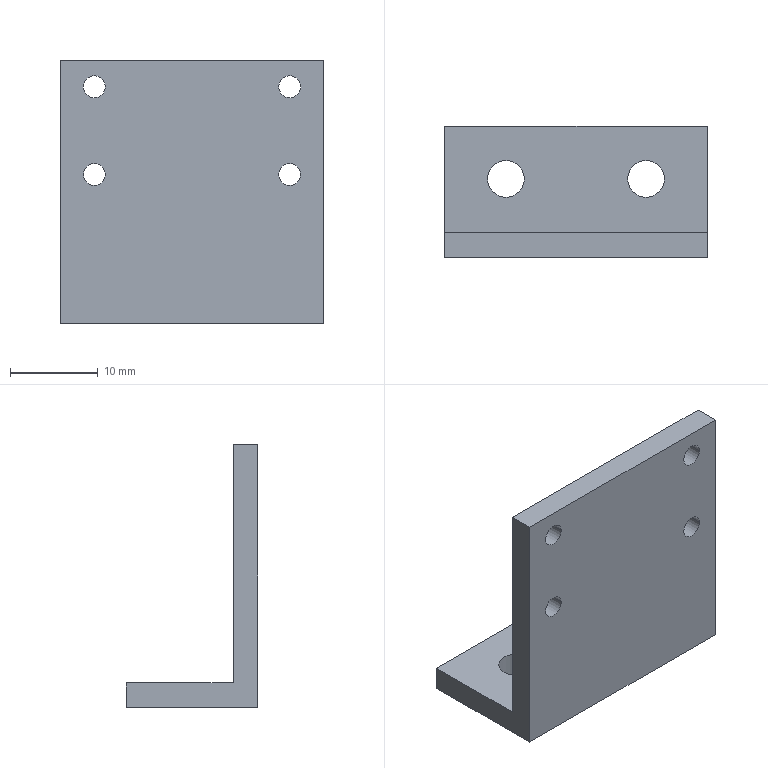Component | SolidWorks | 6G-DCSG-StopSwitchSeat-1 | 1 solid | 20 faces | box 30 x 15 x 30 mm | volume 3412 mm3 | cylinder 12 | plane 8 | commonest cylinder face diameters 2.5 x8 4.2 x4
build123d program:
from build123d import *

# Parameters (mm, degrees)
BOSS_EXTRUDE1_DEPTH = 15
SKETCH2_R           = 2.1
CUT_EXTRUDE1_DEPTH  = 10
M3_TAPPED_HOLE1_D   = 2.5


with BuildPart() as part:
    # Sketch1 → Boss-Extrude1 (new, symmetric)
    with BuildSketch(Plane.XY):
        Polygon((-15, 4.7), (12.2, 4.7), (12.2, -7.5), (15, -7.5), (15, 7.5), (-15, 7.5), align=None)
    extrude(amount=BOSS_EXTRUDE1_DEPTH, both=True)

    # Sketch2 → Cut-Extrude1 (cut)
    with BuildSketch(Plane.ZY.offset(-12.2)):
        with Locations((-8, -1.5)):
            Circle(SKETCH2_R)
        with Locations((8, -1.5)):
            Circle(SKETCH2_R)
    extrude(amount=-CUT_EXTRUDE1_DEPTH, mode=Mode.SUBTRACT)

    # M3 Tapped Hole1 (through all)
    with Locations(Plane(origin=(-12, 4.7, 11.15), x_dir=(0, 0, -1), z_dir=(0, -1, 0))):
        with Locations((0, 0), (0, 10), (22.3, 0), (22.3, 10)):
            Hole(M3_TAPPED_HOLE1_D / 2)


solid = part.part

# Placed as in the assembly
solid = solid.moved(Location((-162, 88.5, 15), (180, -90, 0)))
STEP:
#1=CARTESIAN_POINT('',(-6.866,3.189,1.063));
#2=VERTEX_POINT('',#1);
#3=CARTESIAN_POINT('',(-6.768,3.189,1.063));
#4=VERTEX_POINT('',#3);
#5=CARTESIAN_POINT('',(-6.817,3.189,1.063));
#6=DIRECTION('',(-0.,1.,0.));
#7=DIRECTION('',(1.,0.,0.));
#8=AXIS2_PLACEMENT_3D('',#5,#6,#7);
#9=CIRCLE('',#8,0.04921);
#10=EDGE_CURVE('',#2,#4,#9,.T.);
#11=ORIENTED_EDGE('',*,*,#10,.F.);
#12=CARTESIAN_POINT('',(-6.866,3.299,1.063));
#13=VERTEX_POINT('',#12);
#14=CARTESIAN_POINT('',(-6.866,3.299,1.063));
#15=DIRECTION('',(-0.,1.,0.));
#16=VECTOR('',#15,39.37);
#17=LINE('',#14,#16);
#18=EDGE_CURVE('',#2,#13,#17,.T.);
#19=ORIENTED_EDGE('',*,*,#18,.T.);
#20=CARTESIAN_POINT('',(-6.768,3.299,1.063));
#21=VERTEX_POINT('',#20);
#22=CARTESIAN_POINT('',(-6.817,3.299,1.063));
#23=DIRECTION('',(-0.,1.,0.));
#24=DIRECTION('',(1.,0.,0.));
#25=AXIS2_PLACEMENT_3D('',#22,#23,#24);
#26=CIRCLE('',#25,0.04921);
#27=EDGE_CURVE('',#13,#21,#26,.T.);
#28=ORIENTED_EDGE('',*,*,#27,.T.);
#29=CARTESIAN_POINT('',(-6.768,3.299,1.063));
#30=DIRECTION('',(-0.,1.,0.));
#31=VECTOR('',#30,39.37);
#32=LINE('',#29,#31);
#33=EDGE_CURVE('',#4,#21,#32,.T.);
#34=ORIENTED_EDGE('',*,*,#33,.F.);
#35=EDGE_LOOP('',(#11,#19,#28,#34));
#36=FACE_OUTER_BOUND('',#35,.T.);
#37=CARTESIAN_POINT('',(-6.817,3.299,1.063));
#38=DIRECTION('',(-0.,1.,0.));
#39=DIRECTION('',(1.,0.,0.));
#40=AXIS2_PLACEMENT_3D('',#37,#38,#39);
#41=CYLINDRICAL_SURFACE('',#40,0.04921);
#42=ADVANCED_FACE('',(#36),#41,.F.);
#43=CARTESIAN_POINT('',(-6.866,3.189,0.6693));
#44=VERTEX_POINT('',#43);
#45=CARTESIAN_POINT('',(-6.768,3.189,0.6693));
#46=VERTEX_POINT('',#45);
#47=CARTESIAN_POINT('',(-6.817,3.189,0.6693));
#48=DIRECTION('',(-0.,1.,0.));
#49=DIRECTION('',(1.,0.,0.));
#50=AXIS2_PLACEMENT_3D('',#47,#48,#49);
#51=CIRCLE('',#50,0.04921);
#52=EDGE_CURVE('',#44,#46,#51,.T.);
#53=ORIENTED_EDGE('',*,*,#52,.F.);
#54=CARTESIAN_POINT('',(-6.866,3.299,0.6693));
#55=VERTEX_POINT('',#54);
#56=CARTESIAN_POINT('',(-6.866,3.299,0.6693));
#57=DIRECTION('',(-0.,1.,0.));
#58=VECTOR('',#57,39.37);
#59=LINE('',#56,#58);
#60=EDGE_CURVE('',#44,#55,#59,.T.);
#61=ORIENTED_EDGE('',*,*,#60,.T.);
#62=CARTESIAN_POINT('',(-6.768,3.299,0.6693));
#63=VERTEX_POINT('',#62);
#64=CARTESIAN_POINT('',(-6.817,3.299,0.6693));
#65=DIRECTION('',(-0.,1.,0.));
#66=DIRECTION('',(1.,0.,0.));
#67=AXIS2_PLACEMENT_3D('',#64,#65,#66);
#68=CIRCLE('',#67,0.04921);
#69=EDGE_CURVE('',#55,#63,#68,.T.);
#70=ORIENTED_EDGE('',*,*,#69,.T.);
#71=CARTESIAN_POINT('',(-6.768,3.299,0.6693));
#72=DIRECTION('',(-0.,1.,0.));
#73=VECTOR('',#72,39.37);
#74=LINE('',#71,#73);
#75=EDGE_CURVE('',#46,#63,#74,.T.);
#76=ORIENTED_EDGE('',*,*,#75,.F.);
#77=EDGE_LOOP('',(#53,#61,#70,#76));
#78=FACE_OUTER_BOUND('',#77,.T.);
#79=CARTESIAN_POINT('',(-6.817,3.299,0.6693));
#80=DIRECTION('',(-0.,1.,0.));
#81=DIRECTION('',(1.,0.,0.));
#82=AXIS2_PLACEMENT_3D('',#79,#80,#81);
#83=CYLINDRICAL_SURFACE('',#82,0.04921);
#84=ADVANCED_FACE('',(#78),#83,.F.);
#85=CARTESIAN_POINT('',(-5.988,3.189,1.063));
#86=VERTEX_POINT('',#85);
#87=CARTESIAN_POINT('',(-5.89,3.189,1.063));
#88=VERTEX_POINT('',#87);
#89=CARTESIAN_POINT('',(-5.939,3.189,1.063));
#90=DIRECTION('',(-0.,1.,0.));
#91=DIRECTION('',(1.,0.,0.));
#92=AXIS2_PLACEMENT_3D('',#89,#90,#91);
#93=CIRCLE('',#92,0.04921);
#94=EDGE_CURVE('',#86,#88,#93,.T.);
#95=ORIENTED_EDGE('',*,*,#94,.F.);
#96=CARTESIAN_POINT('',(-5.988,3.299,1.063));
#97=VERTEX_POINT('',#96);
#98=CARTESIAN_POINT('',(-5.988,3.299,1.063));
#99=DIRECTION('',(-0.,1.,0.));
#100=VECTOR('',#99,39.37);
#101=LINE('',#98,#100);
#102=EDGE_CURVE('',#86,#97,#101,.T.);
#103=ORIENTED_EDGE('',*,*,#102,.T.);
#104=CARTESIAN_POINT('',(-5.89,3.299,1.063));
#105=VERTEX_POINT('',#104);
#106=CARTESIAN_POINT('',(-5.939,3.299,1.063));
#107=DIRECTION('',(-0.,1.,0.));
#108=DIRECTION('',(1.,0.,0.));
#109=AXIS2_PLACEMENT_3D('',#106,#107,#108);
#110=CIRCLE('',#109,0.04921);
#111=EDGE_CURVE('',#97,#105,#110,.T.);
#112=ORIENTED_EDGE('',*,*,#111,.T.);
#113=CARTESIAN_POINT('',(-5.89,3.299,1.063));
#114=DIRECTION('',(-0.,1.,0.));
#115=VECTOR('',#114,39.37);
#116=LINE('',#113,#115);
#117=EDGE_CURVE('',#88,#105,#116,.T.);
#118=ORIENTED_EDGE('',*,*,#117,.F.);
#119=EDGE_LOOP('',(#95,#103,#112,#118));
#120=FACE_OUTER_BOUND('',#119,.T.);
#121=CARTESIAN_POINT('',(-5.939,3.299,1.063));
#122=DIRECTION('',(-0.,1.,0.));
#123=DIRECTION('',(1.,0.,0.));
#124=AXIS2_PLACEMENT_3D('',#121,#122,#123);
#125=CYLINDRICAL_SURFACE('',#124,0.04921);
#126=ADVANCED_FACE('',(#120),#125,.F.);
#127=CARTESIAN_POINT('',(-5.988,3.189,0.6693));
#128=VERTEX_POINT('',#127);
#129=CARTESIAN_POINT('',(-5.89,3.189,0.6693));
#130=VERTEX_POINT('',#129);
#131=CARTESIAN_POINT('',(-5.939,3.189,0.6693));
#132=DIRECTION('',(-0.,1.,0.));
#133=DIRECTION('',(1.,0.,0.));
#134=AXIS2_PLACEMENT_3D('',#131,#132,#133);
#135=CIRCLE('',#134,0.04921);
#136=EDGE_CURVE('',#128,#130,#135,.T.);
#137=ORIENTED_EDGE('',*,*,#136,.F.);
#138=CARTESIAN_POINT('',(-5.988,3.299,0.6693));
#139=VERTEX_POINT('',#138);
#140=CARTESIAN_POINT('',(-5.988,3.299,0.6693));
#141=DIRECTION('',(-0.,1.,0.));
#142=VECTOR('',#141,39.37);
#143=LINE('',#140,#142);
#144=EDGE_CURVE('',#128,#139,#143,.T.);
#145=ORIENTED_EDGE('',*,*,#144,.T.);
#146=CARTESIAN_POINT('',(-5.89,3.299,0.6693));
#147=VERTEX_POINT('',#146);
#148=CARTESIAN_POINT('',(-5.939,3.299,0.6693));
#149=DIRECTION('',(-0.,1.,0.));
#150=DIRECTION('',(1.,0.,0.));
#151=AXIS2_PLACEMENT_3D('',#148,#149,#150);
#152=CIRCLE('',#151,0.04921);
#153=EDGE_CURVE('',#139,#147,#152,.T.);
#154=ORIENTED_EDGE('',*,*,#153,.T.);
#155=CARTESIAN_POINT('',(-5.89,3.299,0.6693));
#156=DIRECTION('',(-0.,1.,0.));
#157=VECTOR('',#156,39.37);
#158=LINE('',#155,#157);
#159=EDGE_CURVE('',#130,#147,#158,.T.);
#160=ORIENTED_EDGE('',*,*,#159,.F.);
#161=EDGE_LOOP('',(#137,#145,#154,#160));
#162=FACE_OUTER_BOUND('',#161,.T.);
#163=CARTESIAN_POINT('',(-5.939,3.299,0.6693));
#164=DIRECTION('',(-0.,1.,0.));
#165=DIRECTION('',(1.,0.,0.));
#166=AXIS2_PLACEMENT_3D('',#163,#164,#165);
#167=CYLINDRICAL_SURFACE('',#166,0.04921);
#168=ADVANCED_FACE('',(#162),#167,.F.);
#169=CARTESIAN_POINT('',(-6.61,3.543,0.));
#170=VERTEX_POINT('',#169);
#171=CARTESIAN_POINT('',(-6.776,3.543,0.));
#172=VERTEX_POINT('',#171);
#173=CARTESIAN_POINT('',(-6.693,3.543,0.));
#174=DIRECTION('',(-0.,-0.,1.));
#175=DIRECTION('',(-1.,0.,0.));
#176=AXIS2_PLACEMENT_3D('',#173,#174,#175);
#177=CIRCLE('',#176,0.08268);
#178=EDGE_CURVE('',#170,#172,#177,.T.);
#179=ORIENTED_EDGE('',*,*,#178,.F.);
#180=CARTESIAN_POINT('',(-6.61,3.543,0.1102));
#181=VERTEX_POINT('',#180);
#182=CARTESIAN_POINT('',(-6.61,3.543,-0.2835));
#183=DIRECTION('',(-0.,-0.,1.));
#184=VECTOR('',#183,39.37);
#185=LINE('',#182,#184);
#186=EDGE_CURVE('',#170,#181,#185,.T.);
#187=ORIENTED_EDGE('',*,*,#186,.T.);
#188=CARTESIAN_POINT('',(-6.776,3.543,0.1102));
#189=VERTEX_POINT('',#188);
#190=CARTESIAN_POINT('',(-6.693,3.543,0.1102));
#191=DIRECTION('',(-0.,-0.,1.));
#192=DIRECTION('',(-1.,0.,0.));
#193=AXIS2_PLACEMENT_3D('',#190,#191,#192);
#194=CIRCLE('',#193,0.08268);
#195=EDGE_CURVE('',#181,#189,#194,.T.);
#196=ORIENTED_EDGE('',*,*,#195,.T.);
#197=CARTESIAN_POINT('',(-6.776,3.543,-0.2835));
#198=DIRECTION('',(-0.,-0.,1.));
#199=VECTOR('',#198,39.37);
#200=LINE('',#197,#199);
#201=EDGE_CURVE('',#172,#189,#200,.T.);
#202=ORIENTED_EDGE('',*,*,#201,.F.);
#203=EDGE_LOOP('',(#179,#187,#196,#202));
#204=FACE_OUTER_BOUND('',#203,.T.);
#205=CARTESIAN_POINT('',(-6.693,3.543,-0.2835));
#206=DIRECTION('',(-0.,-0.,1.));
#207=DIRECTION('',(-1.,0.,0.));
#208=AXIS2_PLACEMENT_3D('',#205,#206,#207);
#209=CYLINDRICAL_SURFACE('',#208,0.08268);
#210=ADVANCED_FACE('',(#204),#209,.F.);
#211=CARTESIAN_POINT('',(-5.98,3.543,0.));
#212=VERTEX_POINT('',#211);
#213=CARTESIAN_POINT('',(-6.146,3.543,0.));
#214=VERTEX_POINT('',#213);
#215=CARTESIAN_POINT('',(-6.063,3.543,0.));
#216=DIRECTION('',(-0.,-0.,1.));
#217=DIRECTION('',(-1.,0.,0.));
#218=AXIS2_PLACEMENT_3D('',#215,#216,#217);
#219=CIRCLE('',#218,0.08268);
#220=EDGE_CURVE('',#212,#214,#219,.T.);
#221=ORIENTED_EDGE('',*,*,#220,.F.);
#222=CARTESIAN_POINT('',(-5.98,3.543,0.1102));
#223=VERTEX_POINT('',#222);
#224=CARTESIAN_POINT('',(-5.98,3.543,-0.2835));
#225=DIRECTION('',(-0.,-0.,1.));
#226=VECTOR('',#225,39.37);
#227=LINE('',#224,#226);
#228=EDGE_CURVE('',#212,#223,#227,.T.);
#229=ORIENTED_EDGE('',*,*,#228,.T.);
#230=CARTESIAN_POINT('',(-6.146,3.543,0.1102));
#231=VERTEX_POINT('',#230);
#232=CARTESIAN_POINT('',(-6.063,3.543,0.1102));
#233=DIRECTION('',(-0.,-0.,1.));
#234=DIRECTION('',(-1.,0.,0.));
#235=AXIS2_PLACEMENT_3D('',#232,#233,#234);
#236=CIRCLE('',#235,0.08268);
#237=EDGE_CURVE('',#223,#231,#236,.T.);
#238=ORIENTED_EDGE('',*,*,#237,.T.);
#239=CARTESIAN_POINT('',(-6.146,3.543,-0.2835));
#240=DIRECTION('',(-0.,-0.,1.));
#241=VECTOR('',#240,39.37);
#242=LINE('',#239,#241);
#243=EDGE_CURVE('',#214,#231,#242,.T.);
#244=ORIENTED_EDGE('',*,*,#243,.F.);
#245=EDGE_LOOP('',(#221,#229,#238,#244));
#246=FACE_OUTER_BOUND('',#245,.T.);
#247=CARTESIAN_POINT('',(-6.063,3.543,-0.2835));
#248=DIRECTION('',(-0.,-0.,1.));
#249=DIRECTION('',(-1.,0.,0.));
#250=AXIS2_PLACEMENT_3D('',#247,#248,#249);
#251=CYLINDRICAL_SURFACE('',#250,0.08268);
#252=ADVANCED_FACE('',(#246),#251,.F.);
#253=CARTESIAN_POINT('',(-6.693,3.543,0.));
#254=DIRECTION('',(-0.,-0.,1.));
#255=DIRECTION('',(-1.,0.,0.));
#256=AXIS2_PLACEMENT_3D('',#253,#254,#255);
#257=CIRCLE('',#256,0.08268);
#258=EDGE_CURVE('',#172,#170,#257,.T.);
#259=ORIENTED_EDGE('',*,*,#258,.T.);
#260=ORIENTED_EDGE('',*,*,#178,.T.);
#261=EDGE_LOOP('',(#259,#260));
#262=FACE_BOUND('',#261,.T.);
#263=CARTESIAN_POINT('',(-6.063,3.543,0.));
#264=DIRECTION('',(-0.,-0.,1.));
#265=DIRECTION('',(-1.,0.,0.));
#266=AXIS2_PLACEMENT_3D('',#263,#264,#265);
#267=CIRCLE('',#266,0.08268);
#268=EDGE_CURVE('',#214,#212,#267,.T.);
#269=ORIENTED_EDGE('',*,*,#268,.T.);
#270=ORIENTED_EDGE('',*,*,#220,.T.);
#271=EDGE_LOOP('',(#269,#270));
#272=FACE_BOUND('',#271,.T.);
#273=CARTESIAN_POINT('',(-5.787,3.78,0.));
#274=VERTEX_POINT('',#273);
#275=CARTESIAN_POINT('',(-5.787,3.189,0.));
#276=VERTEX_POINT('',#275);
#277=CARTESIAN_POINT('',(-5.787,3.78,0.));
#278=DIRECTION('',(0.,-1.,-0.));
#279=VECTOR('',#278,39.37);
#280=LINE('',#277,#279);
#281=EDGE_CURVE('',#274,#276,#280,.T.);
#282=ORIENTED_EDGE('',*,*,#281,.T.);
#283=CARTESIAN_POINT('',(-6.969,3.189,0.));
#284=VERTEX_POINT('',#283);
#285=CARTESIAN_POINT('',(-6.969,3.189,0.));
#286=DIRECTION('',(1.,0.,0.));
#287=VECTOR('',#286,39.37);
#288=LINE('',#285,#287);
#289=EDGE_CURVE('',#284,#276,#288,.T.);
#290=ORIENTED_EDGE('',*,*,#289,.F.);
#291=CARTESIAN_POINT('',(-6.969,3.78,0.));
#292=VERTEX_POINT('',#291);
#293=CARTESIAN_POINT('',(-6.969,3.78,0.));
#294=DIRECTION('',(0.,-1.,-0.));
#295=VECTOR('',#294,39.37);
#296=LINE('',#293,#295);
#297=EDGE_CURVE('',#292,#284,#296,.T.);
#298=ORIENTED_EDGE('',*,*,#297,.F.);
#299=CARTESIAN_POINT('',(-6.969,3.78,0.));
#300=DIRECTION('',(1.,0.,0.));
#301=VECTOR('',#300,39.37);
#302=LINE('',#299,#301);
#303=EDGE_CURVE('',#292,#274,#302,.T.);
#304=ORIENTED_EDGE('',*,*,#303,.T.);
#305=EDGE_LOOP('',(#282,#290,#298,#304));
#306=FACE_OUTER_BOUND('',#305,.T.);
#307=CARTESIAN_POINT('',(-6.969,3.78,0.));
#308=DIRECTION('',(0.,-0.,1.));
#309=DIRECTION('',(-1.,-0.,0.));
#310=AXIS2_PLACEMENT_3D('',#307,#308,#309);
#311=PLANE('',#310);
#312=ADVANCED_FACE('',(#262,#272,#306),#311,.F.);
#313=CARTESIAN_POINT('',(-6.817,3.189,1.063));
#314=DIRECTION('',(-0.,1.,0.));
#315=DIRECTION('',(1.,0.,0.));
#316=AXIS2_PLACEMENT_3D('',#313,#314,#315);
#317=CIRCLE('',#316,0.04921);
#318=EDGE_CURVE('',#4,#2,#317,.T.);
#319=ORIENTED_EDGE('',*,*,#318,.T.);
#320=ORIENTED_EDGE('',*,*,#10,.T.);
#321=EDGE_LOOP('',(#319,#320));
#322=FACE_BOUND('',#321,.T.);
#323=CARTESIAN_POINT('',(-6.817,3.189,0.6693));
#324=DIRECTION('',(-0.,1.,0.));
#325=DIRECTION('',(1.,0.,0.));
#326=AXIS2_PLACEMENT_3D('',#323,#324,#325);
#327=CIRCLE('',#326,0.04921);
#328=EDGE_CURVE('',#46,#44,#327,.T.);
#329=ORIENTED_EDGE('',*,*,#328,.T.);
#330=ORIENTED_EDGE('',*,*,#52,.T.);
#331=EDGE_LOOP('',(#329,#330));
#332=FACE_BOUND('',#331,.T.);
#333=CARTESIAN_POINT('',(-5.939,3.189,1.063));
#334=DIRECTION('',(-0.,1.,0.));
#335=DIRECTION('',(1.,0.,0.));
#336=AXIS2_PLACEMENT_3D('',#333,#334,#335);
#337=CIRCLE('',#336,0.04921);
#338=EDGE_CURVE('',#88,#86,#337,.T.);
#339=ORIENTED_EDGE('',*,*,#338,.T.);
#340=ORIENTED_EDGE('',*,*,#94,.T.);
#341=EDGE_LOOP('',(#339,#340));
#342=FACE_BOUND('',#341,.T.);
#343=CARTESIAN_POINT('',(-5.939,3.189,0.6693));
#344=DIRECTION('',(-0.,1.,0.));
#345=DIRECTION('',(1.,0.,0.));
#346=AXIS2_PLACEMENT_3D('',#343,#344,#345);
#347=CIRCLE('',#346,0.04921);
#348=EDGE_CURVE('',#130,#128,#347,.T.);
#349=ORIENTED_EDGE('',*,*,#348,.T.);
#350=ORIENTED_EDGE('',*,*,#136,.T.);
#351=EDGE_LOOP('',(#349,#350));
#352=FACE_BOUND('',#351,.T.);
#353=CARTESIAN_POINT('',(-5.787,3.189,1.181));
#354=VERTEX_POINT('',#353);
#355=CARTESIAN_POINT('',(-5.787,3.189,1.181));
#356=DIRECTION('',(-0.,-0.,1.));
#357=VECTOR('',#356,39.37);
#358=LINE('',#355,#357);
#359=EDGE_CURVE('',#276,#354,#358,.T.);
#360=ORIENTED_EDGE('',*,*,#359,.T.);
#361=CARTESIAN_POINT('',(-6.969,3.189,1.181));
#362=VERTEX_POINT('',#361);
#363=CARTESIAN_POINT('',(-6.969,3.189,1.181));
#364=DIRECTION('',(1.,0.,0.));
#365=VECTOR('',#364,39.37);
#366=LINE('',#363,#365);
#367=EDGE_CURVE('',#362,#354,#366,.T.);
#368=ORIENTED_EDGE('',*,*,#367,.F.);
#369=CARTESIAN_POINT('',(-6.969,3.189,1.181));
#370=DIRECTION('',(-0.,-0.,1.));
#371=VECTOR('',#370,39.37);
#372=LINE('',#369,#371);
#373=EDGE_CURVE('',#284,#362,#372,.T.);
#374=ORIENTED_EDGE('',*,*,#373,.F.);
#375=ORIENTED_EDGE('',*,*,#289,.T.);
#376=EDGE_LOOP('',(#360,#368,#374,#375));
#377=FACE_OUTER_BOUND('',#376,.T.);
#378=CARTESIAN_POINT('',(-6.969,3.189,1.181));
#379=DIRECTION('',(-0.,1.,0.));
#380=DIRECTION('',(1.,0.,0.));
#381=AXIS2_PLACEMENT_3D('',#378,#379,#380);
#382=PLANE('',#381);
#383=ADVANCED_FACE('',(#322,#332,#342,#352,#377),#382,.F.);
#384=CARTESIAN_POINT('',(-5.787,3.299,1.181));
#385=VERTEX_POINT('',#384);
#386=CARTESIAN_POINT('',(-5.787,3.299,1.181));
#387=DIRECTION('',(-0.,1.,0.));
#388=VECTOR('',#387,39.37);
#389=LINE('',#386,#388);
#390=EDGE_CURVE('',#354,#385,#389,.T.);
#391=ORIENTED_EDGE('',*,*,#390,.T.);
#392=CARTESIAN_POINT('',(-6.969,3.299,1.181));
#393=VERTEX_POINT('',#392);
#394=CARTESIAN_POINT('',(-6.969,3.299,1.181));
#395=DIRECTION('',(1.,0.,0.));
#396=VECTOR('',#395,39.37);
#397=LINE('',#394,#396);
#398=EDGE_CURVE('',#393,#385,#397,.T.);
#399=ORIENTED_EDGE('',*,*,#398,.F.);
#400=CARTESIAN_POINT('',(-6.969,3.299,1.181));
#401=DIRECTION('',(-0.,1.,0.));
#402=VECTOR('',#401,39.37);
#403=LINE('',#400,#402);
#404=EDGE_CURVE('',#362,#393,#403,.T.);
#405=ORIENTED_EDGE('',*,*,#404,.F.);
#406=ORIENTED_EDGE('',*,*,#367,.T.);
#407=EDGE_LOOP('',(#391,#399,#405,#406));
#408=FACE_OUTER_BOUND('',#407,.T.);
#409=CARTESIAN_POINT('',(-6.969,3.299,1.181));
#410=DIRECTION('',(-0.,0.,-1.));
#411=DIRECTION('',(1.,0.,0.));
#412=AXIS2_PLACEMENT_3D('',#409,#410,#411);
#413=PLANE('',#412);
#414=ADVANCED_FACE('',(#408),#413,.F.);
#415=CARTESIAN_POINT('',(-6.817,3.299,1.063));
#416=DIRECTION('',(-0.,1.,0.));
#417=DIRECTION('',(1.,0.,0.));
#418=AXIS2_PLACEMENT_3D('',#415,#416,#417);
#419=CIRCLE('',#418,0.04921);
#420=EDGE_CURVE('',#21,#13,#419,.T.);
#421=ORIENTED_EDGE('',*,*,#420,.F.);
#422=ORIENTED_EDGE('',*,*,#27,.F.);
#423=EDGE_LOOP('',(#421,#422));
#424=FACE_BOUND('',#423,.T.);
#425=CARTESIAN_POINT('',(-6.817,3.299,0.6693));
#426=DIRECTION('',(-0.,1.,0.));
#427=DIRECTION('',(1.,0.,0.));
#428=AXIS2_PLACEMENT_3D('',#425,#426,#427);
#429=CIRCLE('',#428,0.04921);
#430=EDGE_CURVE('',#63,#55,#429,.T.);
#431=ORIENTED_EDGE('',*,*,#430,.F.);
#432=ORIENTED_EDGE('',*,*,#69,.F.);
#433=EDGE_LOOP('',(#431,#432));
#434=FACE_BOUND('',#433,.T.);
#435=CARTESIAN_POINT('',(-5.939,3.299,1.063));
#436=DIRECTION('',(-0.,1.,0.));
#437=DIRECTION('',(1.,0.,0.));
#438=AXIS2_PLACEMENT_3D('',#435,#436,#437);
#439=CIRCLE('',#438,0.04921);
#440=EDGE_CURVE('',#105,#97,#439,.T.);
#441=ORIENTED_EDGE('',*,*,#440,.F.);
#442=ORIENTED_EDGE('',*,*,#111,.F.);
#443=EDGE_LOOP('',(#441,#442));
#444=FACE_BOUND('',#443,.T.);
#445=CARTESIAN_POINT('',(-5.939,3.299,0.6693));
#446=DIRECTION('',(-0.,1.,0.));
#447=DIRECTION('',(1.,0.,0.));
#448=AXIS2_PLACEMENT_3D('',#445,#446,#447);
#449=CIRCLE('',#448,0.04921);
#450=EDGE_CURVE('',#147,#139,#449,.T.);
#451=ORIENTED_EDGE('',*,*,#450,.F.);
#452=ORIENTED_EDGE('',*,*,#153,.F.);
#453=EDGE_LOOP('',(#451,#452));
#454=FACE_BOUND('',#453,.T.);
#455=CARTESIAN_POINT('',(-5.787,3.299,0.1102));
#456=VERTEX_POINT('',#455);
#457=CARTESIAN_POINT('',(-5.787,3.299,1.181));
#458=DIRECTION('',(0.,0.,-1.));
#459=VECTOR('',#458,39.37);
#460=LINE('',#457,#459);
#461=EDGE_CURVE('',#385,#456,#460,.T.);
#462=ORIENTED_EDGE('',*,*,#461,.T.);
#463=CARTESIAN_POINT('',(-6.969,3.299,0.1102));
#464=VERTEX_POINT('',#463);
#465=CARTESIAN_POINT('',(-6.969,3.299,0.1102));
#466=DIRECTION('',(1.,0.,0.));
#467=VECTOR('',#466,39.37);
#468=LINE('',#465,#467);
#469=EDGE_CURVE('',#464,#456,#468,.T.);
#470=ORIENTED_EDGE('',*,*,#469,.F.);
#471=CARTESIAN_POINT('',(-6.969,3.299,1.181));
#472=DIRECTION('',(0.,0.,-1.));
#473=VECTOR('',#472,39.37);
#474=LINE('',#471,#473);
#475=EDGE_CURVE('',#393,#464,#474,.T.);
#476=ORIENTED_EDGE('',*,*,#475,.F.);
#477=ORIENTED_EDGE('',*,*,#398,.T.);
#478=EDGE_LOOP('',(#462,#470,#476,#477));
#479=FACE_OUTER_BOUND('',#478,.T.);
#480=CARTESIAN_POINT('',(-6.969,3.299,1.181));
#481=DIRECTION('',(0.,-1.,-0.));
#482=DIRECTION('',(-1.,-0.,0.));
#483=AXIS2_PLACEMENT_3D('',#480,#481,#482);
#484=PLANE('',#483);
#485=ADVANCED_FACE('',(#424,#434,#444,#454,#479),#484,.F.);
#486=CARTESIAN_POINT('',(-6.693,3.543,0.1102));
#487=DIRECTION('',(-0.,-0.,1.));
#488=DIRECTION('',(-1.,0.,0.));
#489=AXIS2_PLACEMENT_3D('',#486,#487,#488);
#490=CIRCLE('',#489,0.08268);
#491=EDGE_CURVE('',#189,#181,#490,.T.);
#492=ORIENTED_EDGE('',*,*,#491,.F.);
#493=ORIENTED_EDGE('',*,*,#195,.F.);
#494=EDGE_LOOP('',(#492,#493));
#495=FACE_BOUND('',#494,.T.);
#496=CARTESIAN_POINT('',(-6.063,3.543,0.1102));
#497=DIRECTION('',(-0.,-0.,1.));
#498=DIRECTION('',(-1.,0.,0.));
#499=AXIS2_PLACEMENT_3D('',#496,#497,#498);
#500=CIRCLE('',#499,0.08268);
#501=EDGE_CURVE('',#231,#223,#500,.T.);
#502=ORIENTED_EDGE('',*,*,#501,.F.);
#503=ORIENTED_EDGE('',*,*,#237,.F.);
#504=EDGE_LOOP('',(#502,#503));
#505=FACE_BOUND('',#504,.T.);
#506=CARTESIAN_POINT('',(-5.787,3.78,0.1102));
#507=VERTEX_POINT('',#506);
#508=CARTESIAN_POINT('',(-5.787,3.78,0.1102));
#509=DIRECTION('',(-0.,1.,0.));
#510=VECTOR('',#509,39.37);
#511=LINE('',#508,#510);
#512=EDGE_CURVE('',#456,#507,#511,.T.);
#513=ORIENTED_EDGE('',*,*,#512,.T.);
#514=CARTESIAN_POINT('',(-6.969,3.78,0.1102));
#515=VERTEX_POINT('',#514);
#516=CARTESIAN_POINT('',(-6.969,3.78,0.1102));
#517=DIRECTION('',(1.,0.,0.));
#518=VECTOR('',#517,39.37);
#519=LINE('',#516,#518);
#520=EDGE_CURVE('',#515,#507,#519,.T.);
#521=ORIENTED_EDGE('',*,*,#520,.F.);
#522=CARTESIAN_POINT('',(-6.969,3.78,0.1102));
#523=DIRECTION('',(-0.,1.,0.));
#524=VECTOR('',#523,39.37);
#525=LINE('',#522,#524);
#526=EDGE_CURVE('',#464,#515,#525,.T.);
#527=ORIENTED_EDGE('',*,*,#526,.F.);
#528=ORIENTED_EDGE('',*,*,#469,.T.);
#529=EDGE_LOOP('',(#513,#521,#527,#528));
#530=FACE_OUTER_BOUND('',#529,.T.);
#531=CARTESIAN_POINT('',(-6.969,3.78,0.1102));
#532=DIRECTION('',(-0.,0.,-1.));
#533=DIRECTION('',(1.,0.,0.));
#534=AXIS2_PLACEMENT_3D('',#531,#532,#533);
#535=PLANE('',#534);
#536=ADVANCED_FACE('',(#495,#505,#530),#535,.F.);
#537=CARTESIAN_POINT('',(-5.787,3.78,0.1102));
#538=DIRECTION('',(0.,0.,-1.));
#539=VECTOR('',#538,39.37);
#540=LINE('',#537,#539);
#541=EDGE_CURVE('',#507,#274,#540,.T.);
#542=ORIENTED_EDGE('',*,*,#541,.T.);
#543=ORIENTED_EDGE('',*,*,#303,.F.);
#544=CARTESIAN_POINT('',(-6.969,3.78,0.1102));
#545=DIRECTION('',(0.,0.,-1.));
#546=VECTOR('',#545,39.37);
#547=LINE('',#544,#546);
#548=EDGE_CURVE('',#515,#292,#547,.T.);
#549=ORIENTED_EDGE('',*,*,#548,.F.);
#550=ORIENTED_EDGE('',*,*,#520,.T.);
#551=EDGE_LOOP('',(#542,#543,#549,#550));
#552=FACE_OUTER_BOUND('',#551,.T.);
#553=CARTESIAN_POINT('',(-6.969,3.78,0.1102));
#554=DIRECTION('',(0.,-1.,-0.));
#555=DIRECTION('',(-1.,-0.,0.));
#556=AXIS2_PLACEMENT_3D('',#553,#554,#555);
#557=PLANE('',#556);
#558=ADVANCED_FACE('',(#552),#557,.F.);
#559=ORIENTED_EDGE('',*,*,#297,.T.);
#560=ORIENTED_EDGE('',*,*,#373,.T.);
#561=ORIENTED_EDGE('',*,*,#404,.T.);
#562=ORIENTED_EDGE('',*,*,#475,.T.);
#563=ORIENTED_EDGE('',*,*,#526,.T.);
#564=ORIENTED_EDGE('',*,*,#548,.T.);
#565=EDGE_LOOP('',(#559,#560,#561,#562,#563,#564));
#566=FACE_OUTER_BOUND('',#565,.T.);
#567=CARTESIAN_POINT('',(-6.969,3.484,0.5906));
#568=DIRECTION('',(1.,0.,0.));
#569=DIRECTION('',(-0.,-0.,1.));
#570=AXIS2_PLACEMENT_3D('',#567,#568,#569);
#571=PLANE('',#570);
#572=ADVANCED_FACE('',(#566),#571,.F.);
#573=ORIENTED_EDGE('',*,*,#281,.F.);
#574=ORIENTED_EDGE('',*,*,#541,.F.);
#575=ORIENTED_EDGE('',*,*,#512,.F.);
#576=ORIENTED_EDGE('',*,*,#461,.F.);
#577=ORIENTED_EDGE('',*,*,#390,.F.);
#578=ORIENTED_EDGE('',*,*,#359,.F.);
#579=EDGE_LOOP('',(#573,#574,#575,#576,#577,#578));
#580=FACE_OUTER_BOUND('',#579,.T.);
#581=CARTESIAN_POINT('',(-5.787,3.484,0.5906));
#582=DIRECTION('',(1.,0.,0.));
#583=DIRECTION('',(-0.,-0.,1.));
#584=AXIS2_PLACEMENT_3D('',#581,#582,#583);
#585=PLANE('',#584);
#586=ADVANCED_FACE('',(#580),#585,.T.);
#587=ORIENTED_EDGE('',*,*,#228,.F.);
#588=ORIENTED_EDGE('',*,*,#268,.F.);
#589=ORIENTED_EDGE('',*,*,#243,.T.);
#590=ORIENTED_EDGE('',*,*,#501,.T.);
#591=EDGE_LOOP('',(#587,#588,#589,#590));
#592=FACE_OUTER_BOUND('',#591,.T.);
#593=CARTESIAN_POINT('',(-6.063,3.543,-0.2835));
#594=DIRECTION('',(-0.,-0.,1.));
#595=DIRECTION('',(-1.,0.,0.));
#596=AXIS2_PLACEMENT_3D('',#593,#594,#595);
#597=CYLINDRICAL_SURFACE('',#596,0.08268);
#598=ADVANCED_FACE('',(#592),#597,.F.);
#599=ORIENTED_EDGE('',*,*,#186,.F.);
#600=ORIENTED_EDGE('',*,*,#258,.F.);
#601=ORIENTED_EDGE('',*,*,#201,.T.);
#602=ORIENTED_EDGE('',*,*,#491,.T.);
#603=EDGE_LOOP('',(#599,#600,#601,#602));
#604=FACE_OUTER_BOUND('',#603,.T.);
#605=CARTESIAN_POINT('',(-6.693,3.543,-0.2835));
#606=DIRECTION('',(-0.,-0.,1.));
#607=DIRECTION('',(-1.,0.,0.));
#608=AXIS2_PLACEMENT_3D('',#605,#606,#607);
#609=CYLINDRICAL_SURFACE('',#608,0.08268);
#610=ADVANCED_FACE('',(#604),#609,.F.);
#611=ORIENTED_EDGE('',*,*,#144,.F.);
#612=ORIENTED_EDGE('',*,*,#348,.F.);
#613=ORIENTED_EDGE('',*,*,#159,.T.);
#614=ORIENTED_EDGE('',*,*,#450,.T.);
#615=EDGE_LOOP('',(#611,#612,#613,#614));
#616=FACE_OUTER_BOUND('',#615,.T.);
#617=CARTESIAN_POINT('',(-5.939,3.299,0.6693));
#618=DIRECTION('',(-0.,1.,0.));
#619=DIRECTION('',(1.,0.,0.));
#620=AXIS2_PLACEMENT_3D('',#617,#618,#619);
#621=CYLINDRICAL_SURFACE('',#620,0.04921);
#622=ADVANCED_FACE('',(#616),#621,.F.);
#623=ORIENTED_EDGE('',*,*,#102,.F.);
#624=ORIENTED_EDGE('',*,*,#338,.F.);
#625=ORIENTED_EDGE('',*,*,#117,.T.);
#626=ORIENTED_EDGE('',*,*,#440,.T.);
#627=EDGE_LOOP('',(#623,#624,#625,#626));
#628=FACE_OUTER_BOUND('',#627,.T.);
#629=CARTESIAN_POINT('',(-5.939,3.299,1.063));
#630=DIRECTION('',(-0.,1.,0.));
#631=DIRECTION('',(1.,0.,0.));
#632=AXIS2_PLACEMENT_3D('',#629,#630,#631);
#633=CYLINDRICAL_SURFACE('',#632,0.04921);
#634=ADVANCED_FACE('',(#628),#633,.F.);
#635=ORIENTED_EDGE('',*,*,#60,.F.);
#636=ORIENTED_EDGE('',*,*,#328,.F.);
#637=ORIENTED_EDGE('',*,*,#75,.T.);
#638=ORIENTED_EDGE('',*,*,#430,.T.);
#639=EDGE_LOOP('',(#635,#636,#637,#638));
#640=FACE_OUTER_BOUND('',#639,.T.);
#641=CARTESIAN_POINT('',(-6.817,3.299,0.6693));
#642=DIRECTION('',(-0.,1.,0.));
#643=DIRECTION('',(1.,0.,0.));
#644=AXIS2_PLACEMENT_3D('',#641,#642,#643);
#645=CYLINDRICAL_SURFACE('',#644,0.04921);
#646=ADVANCED_FACE('',(#640),#645,.F.);
#647=ORIENTED_EDGE('',*,*,#18,.F.);
#648=ORIENTED_EDGE('',*,*,#318,.F.);
#649=ORIENTED_EDGE('',*,*,#33,.T.);
#650=ORIENTED_EDGE('',*,*,#420,.T.);
#651=EDGE_LOOP('',(#647,#648,#649,#650));
#652=FACE_OUTER_BOUND('',#651,.T.);
#653=CARTESIAN_POINT('',(-6.817,3.299,1.063));
#654=DIRECTION('',(-0.,1.,0.));
#655=DIRECTION('',(1.,0.,0.));
#656=AXIS2_PLACEMENT_3D('',#653,#654,#655);
#657=CYLINDRICAL_SURFACE('',#656,0.04921);
#658=ADVANCED_FACE('',(#652),#657,.F.);
#659=CLOSED_SHELL('',(#42,#84,#126,#168,#210,#252,#312,#383,#414,#485,#536,#558,#572,#586,#598,#610,#622,#634,#646,#658));
#660=MANIFOLD_SOLID_BREP('',#659);
#661=CARTESIAN_POINT('',(0.,0.,0.));
#662=DIRECTION('',(0.,0.,1.));
#663=DIRECTION('',(1.,0.,0.));
#664=AXIS2_PLACEMENT_3D('',#661,#662,#663);
#665=(LENGTH_UNIT()NAMED_UNIT(*)SI_UNIT($,.METRE.));
#666=LENGTH_MEASURE_WITH_UNIT(LENGTH_MEASURE(0.0254),#665);
#667=DIMENSIONAL_EXPONENTS(1.,0.,0.,0.,0.,0.,0.);
#668=(CONVERSION_BASED_UNIT('',#666)LENGTH_UNIT()NAMED_UNIT(#667));
#669=UNCERTAINTY_MEASURE_WITH_UNIT(LENGTH_MEASURE(0.00001),#668,'','');
#670=(NAMED_UNIT(*)PLANE_ANGLE_UNIT()SI_UNIT($,.RADIAN.));
#671=(NAMED_UNIT(*)SI_UNIT($,.STERADIAN.)SOLID_ANGLE_UNIT());
#672=(GEOMETRIC_REPRESENTATION_CONTEXT(3)GLOBAL_UNCERTAINTY_ASSIGNED_CONTEXT((#669))GLOBAL_UNIT_ASSIGNED_CONTEXT((#668,#670,#671))REPRESENTATION_CONTEXT('',''));
#673=ADVANCED_BREP_SHAPE_REPRESENTATION('',(#660,#664),#672);
#674=COLOUR_RGB('',0.7922,0.8196,0.9333);
#675=FILL_AREA_STYLE_COLOUR('',#674);
#676=FILL_AREA_STYLE('',(#675));
#677=SURFACE_STYLE_FILL_AREA(#676);
#678=SURFACE_SIDE_STYLE('',(#677));
#679=SURFACE_STYLE_USAGE(.BOTH.,#678);
#680=PRESENTATION_STYLE_ASSIGNMENT((#679));
#681=STYLED_ITEM('',(#680),#660);
#682=(LENGTH_UNIT()NAMED_UNIT(*)SI_UNIT($,.METRE.));
#683=LENGTH_MEASURE_WITH_UNIT(LENGTH_MEASURE(0.0254),#682);
#684=DIMENSIONAL_EXPONENTS(1.,0.,0.,0.,0.,0.,0.);
#685=(CONVERSION_BASED_UNIT('',#683)LENGTH_UNIT()NAMED_UNIT(#684));
#686=UNCERTAINTY_MEASURE_WITH_UNIT(LENGTH_MEASURE(0.00001),#685,'','');
#687=(NAMED_UNIT(*)PLANE_ANGLE_UNIT()SI_UNIT($,.RADIAN.));
#688=(NAMED_UNIT(*)SI_UNIT($,.STERADIAN.)SOLID_ANGLE_UNIT());
#689=(GEOMETRIC_REPRESENTATION_CONTEXT(3)GLOBAL_UNCERTAINTY_ASSIGNED_CONTEXT((#686))GLOBAL_UNIT_ASSIGNED_CONTEXT((#685,#687,#688))REPRESENTATION_CONTEXT('',''));
#690=MECHANICAL_DESIGN_GEOMETRIC_PRESENTATION_REPRESENTATION('',(#681),#689);
#691=PRESENTATION_LAYER_ASSIGNMENT('','',(#681));